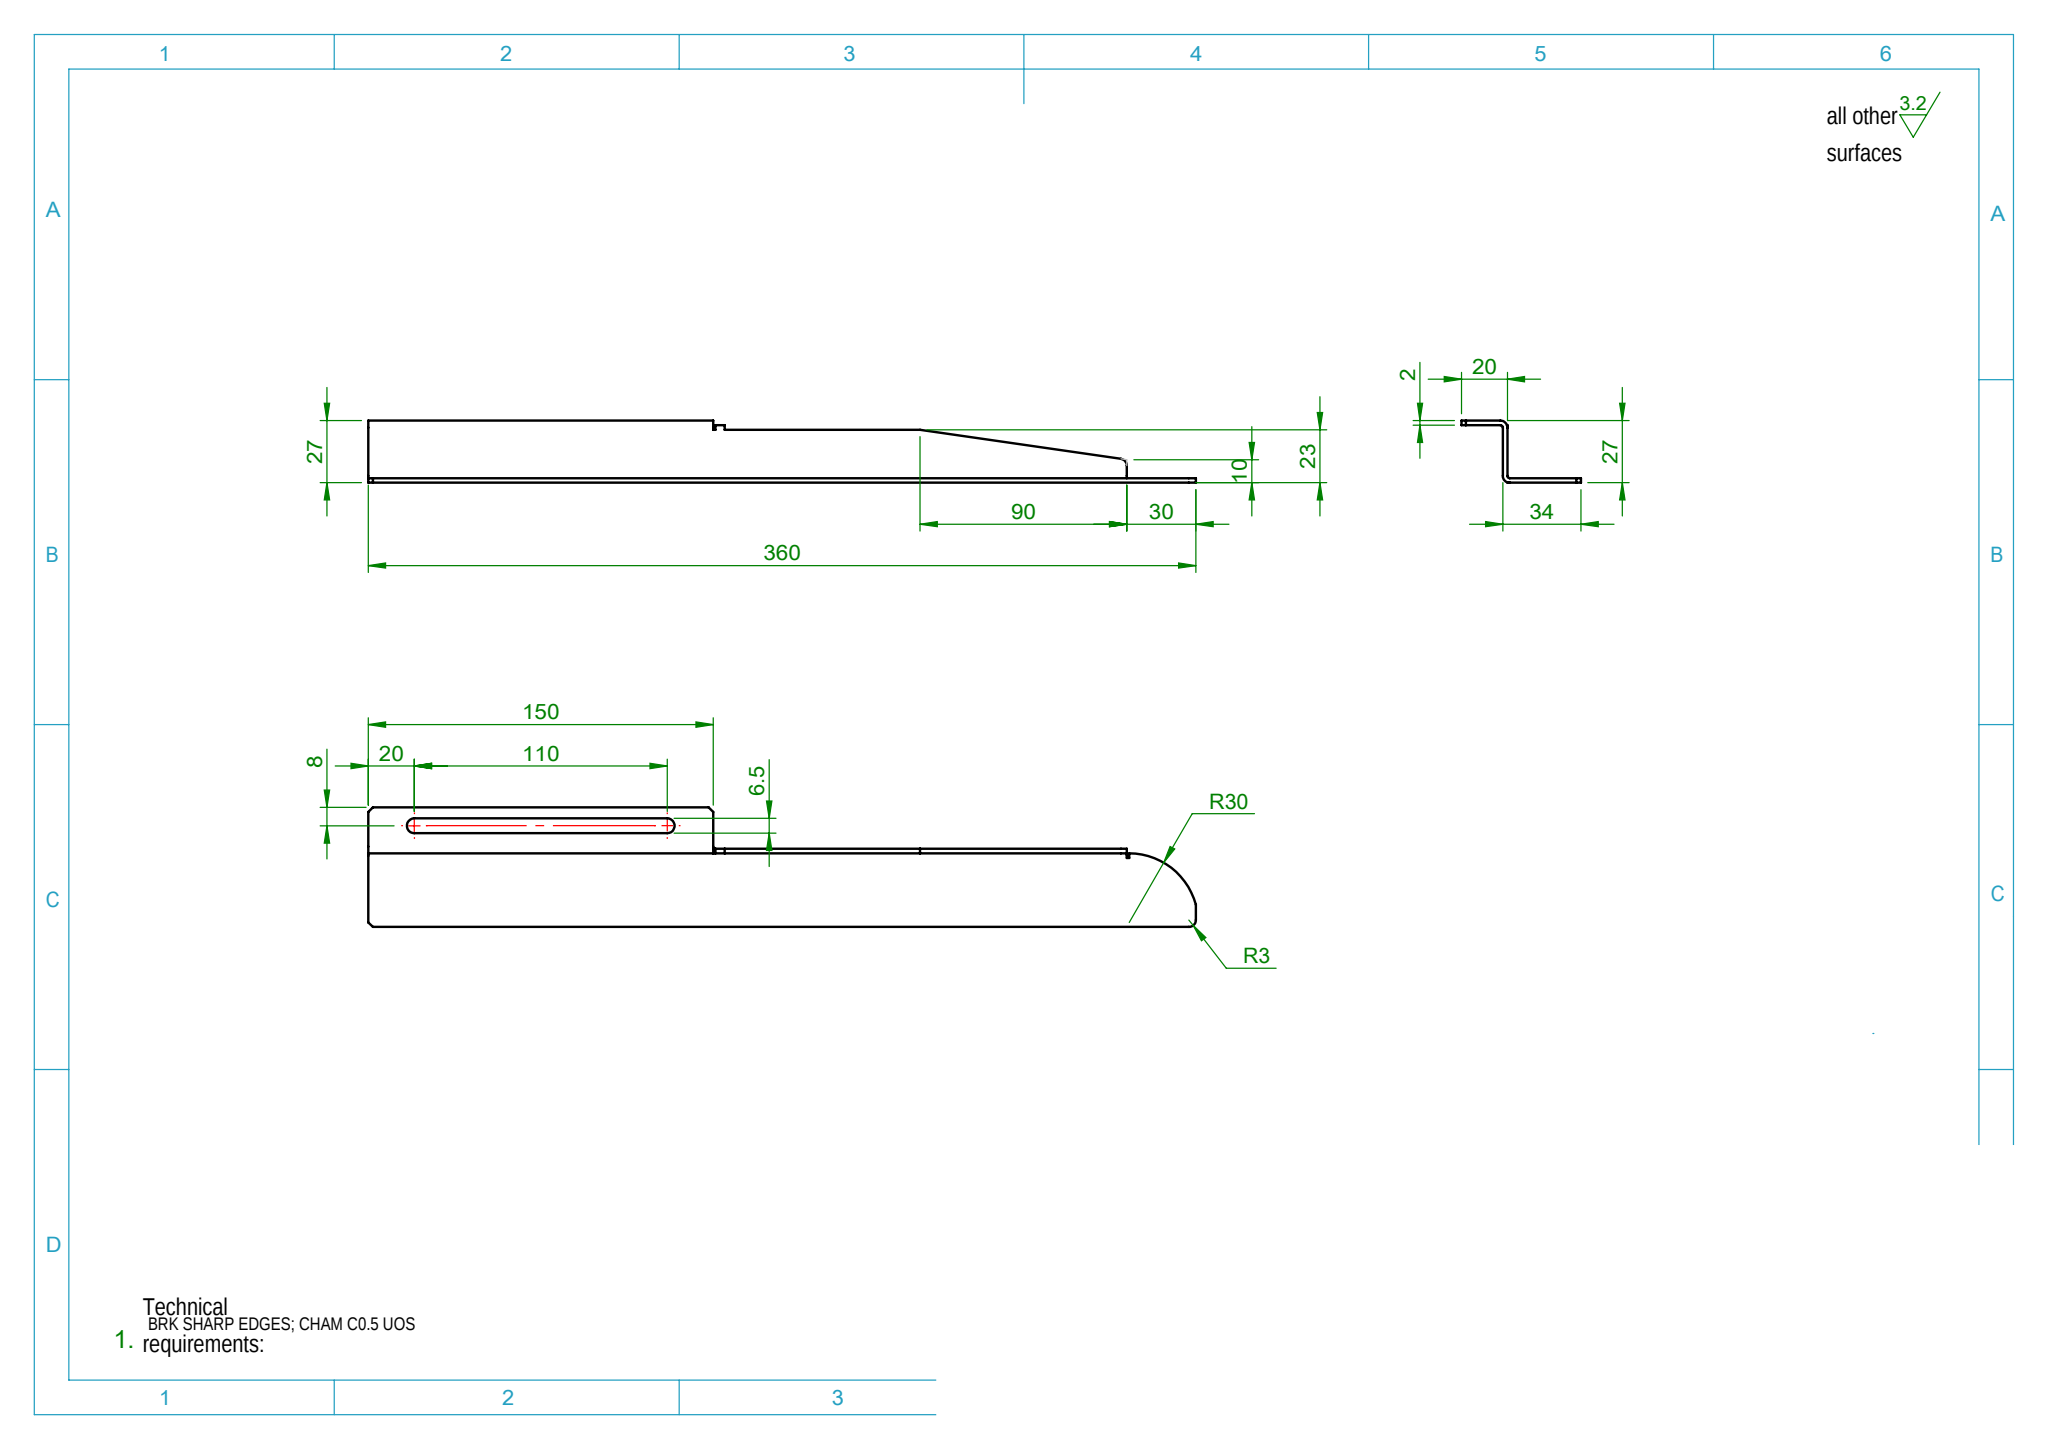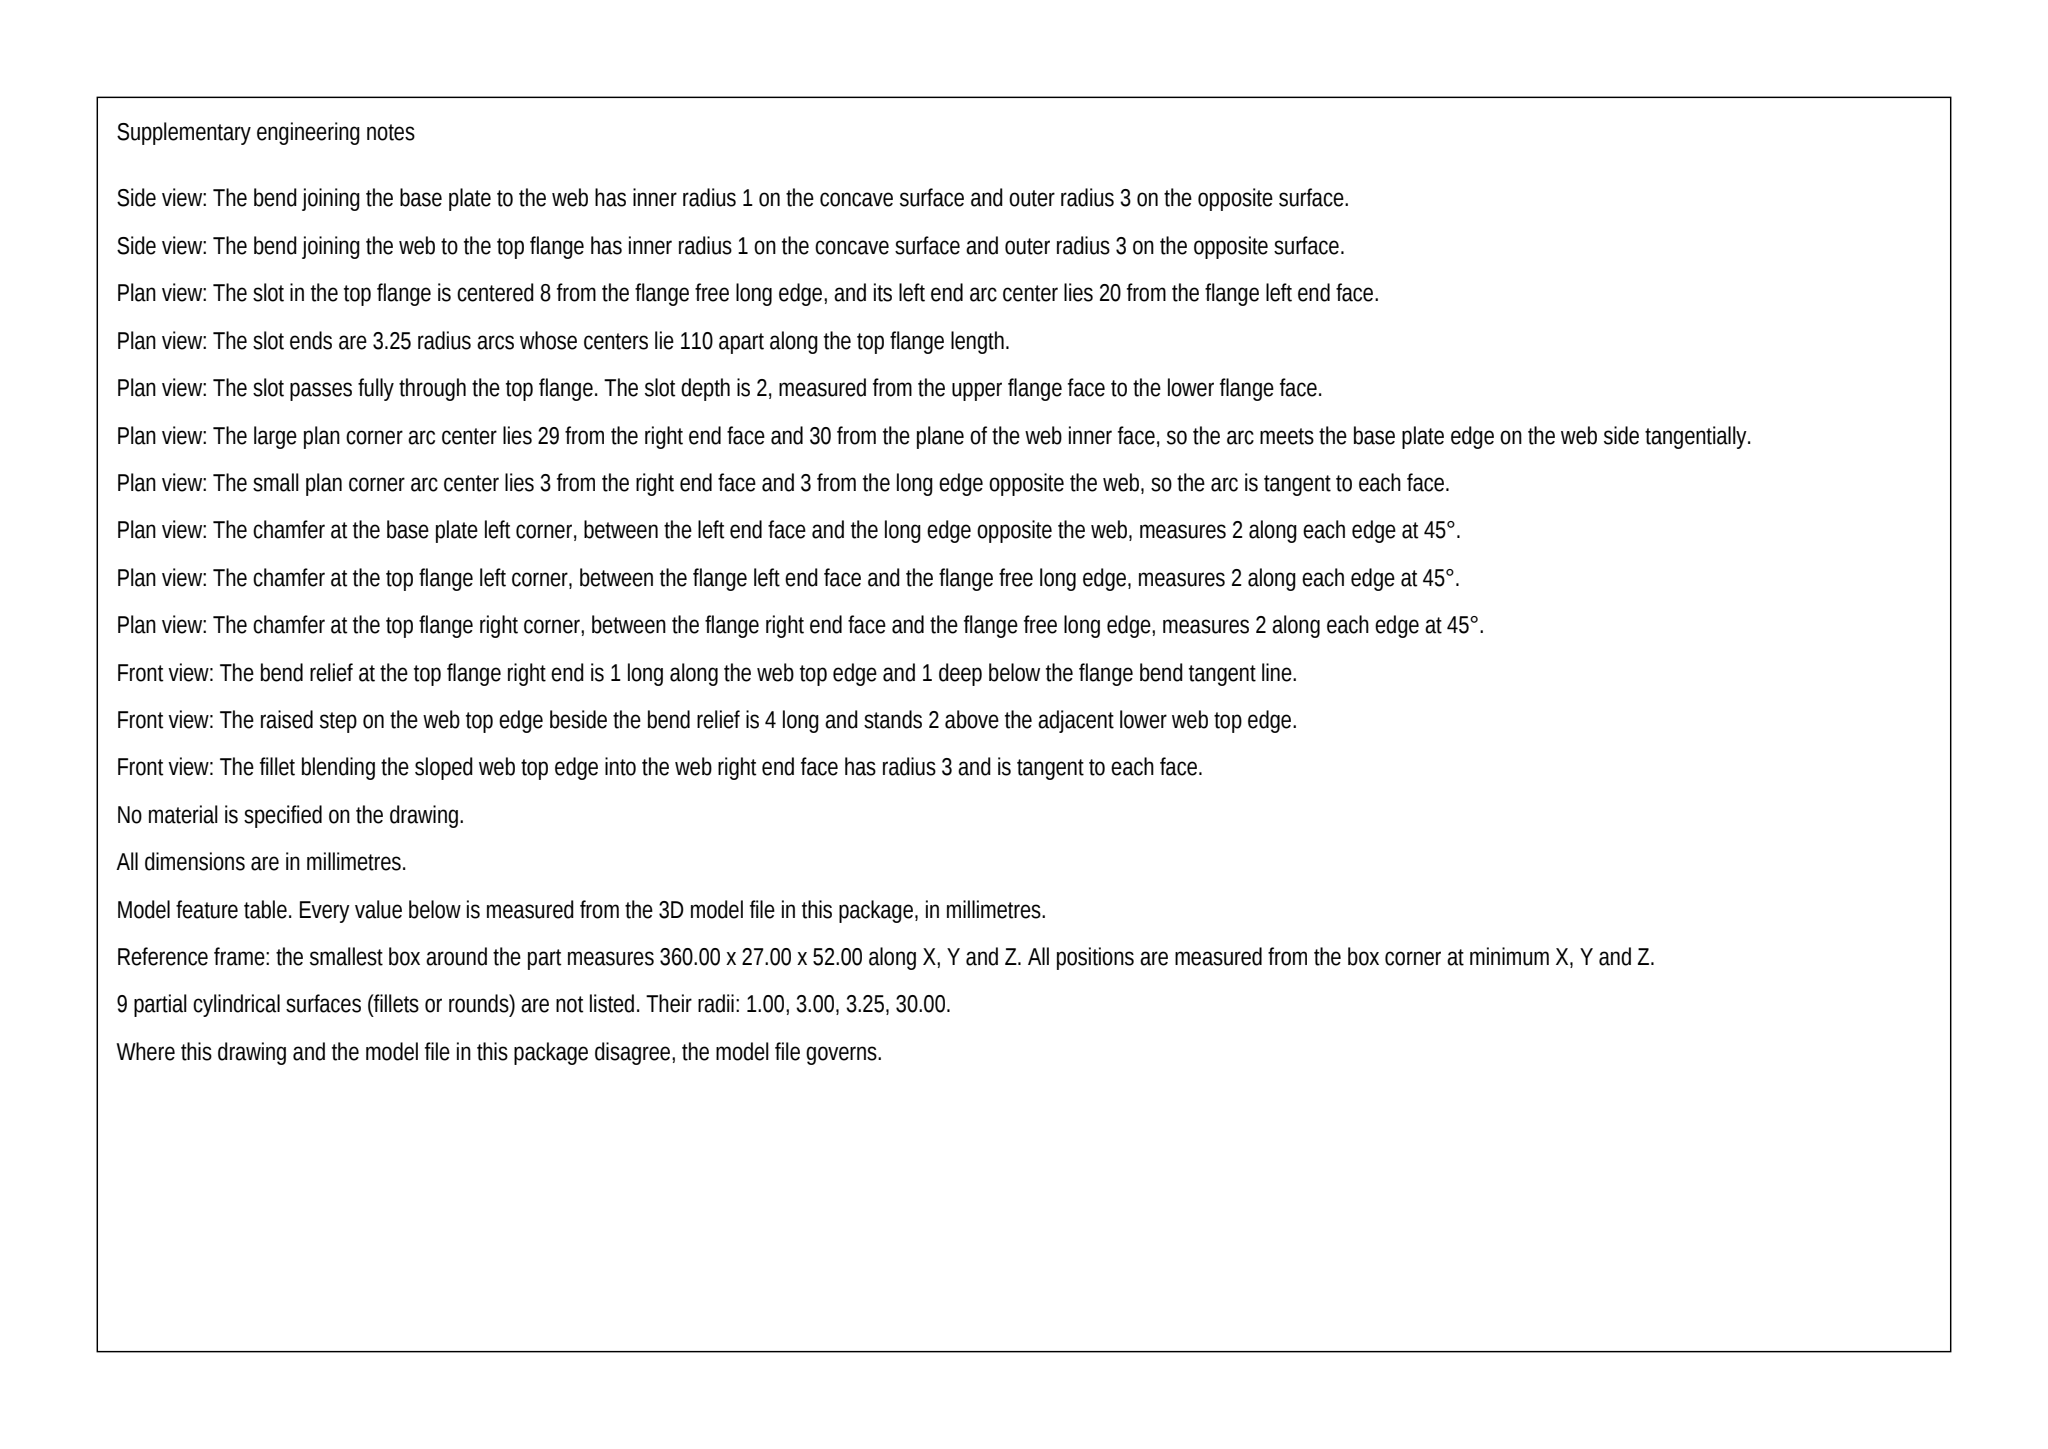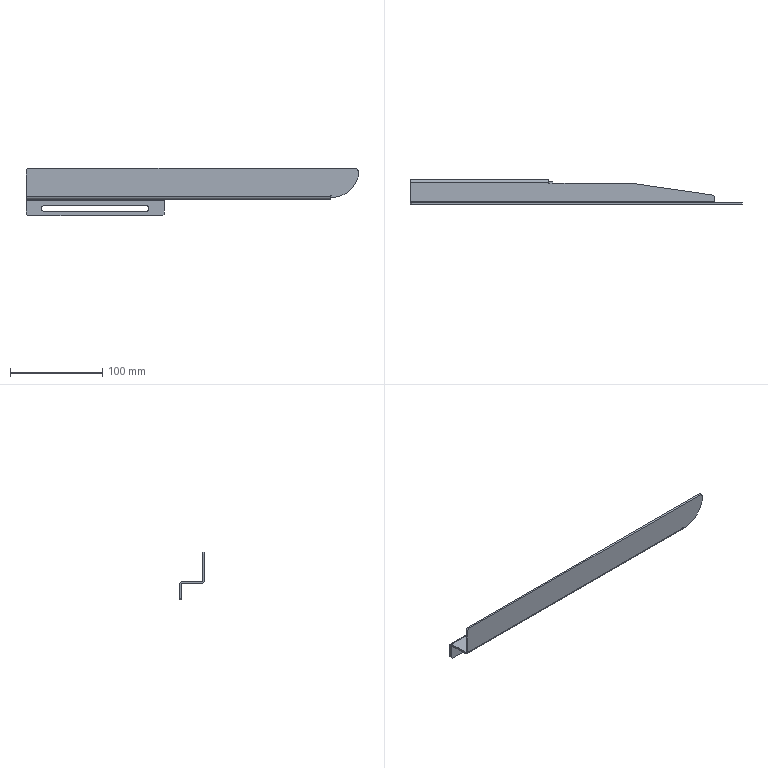Part | SolidWorks | mm | 1 solid | 42 faces | box 360 x 27 x 52 mm | volume 40986 mm3 | plane 33 | cylinder 9 | commonest cylinder face diameters 6 x4 2 x2 6.5 x2 60 x1
Drawing notes:
ALL BENDS R1 INNER (R3 OUTER), MATL 2 THK | from the solid: cyl dia2 (R1) & dia6 (R3) on x-axis at y3/z21 L330 and y24/z17 L150
STEP AT TOP FLANGE END: 4 LG x 4 DEEP, 151 FROM LEFT END | from the solid: x-planes 151 & 155, y-planes 23 & 27 (web 27->23), z=22 face
FRONT VIEW: R3 AT TAPER/10 HIGH END JUNCTION | from the solid: cyl dia6 z-axis at x=327, y=7.4, L2